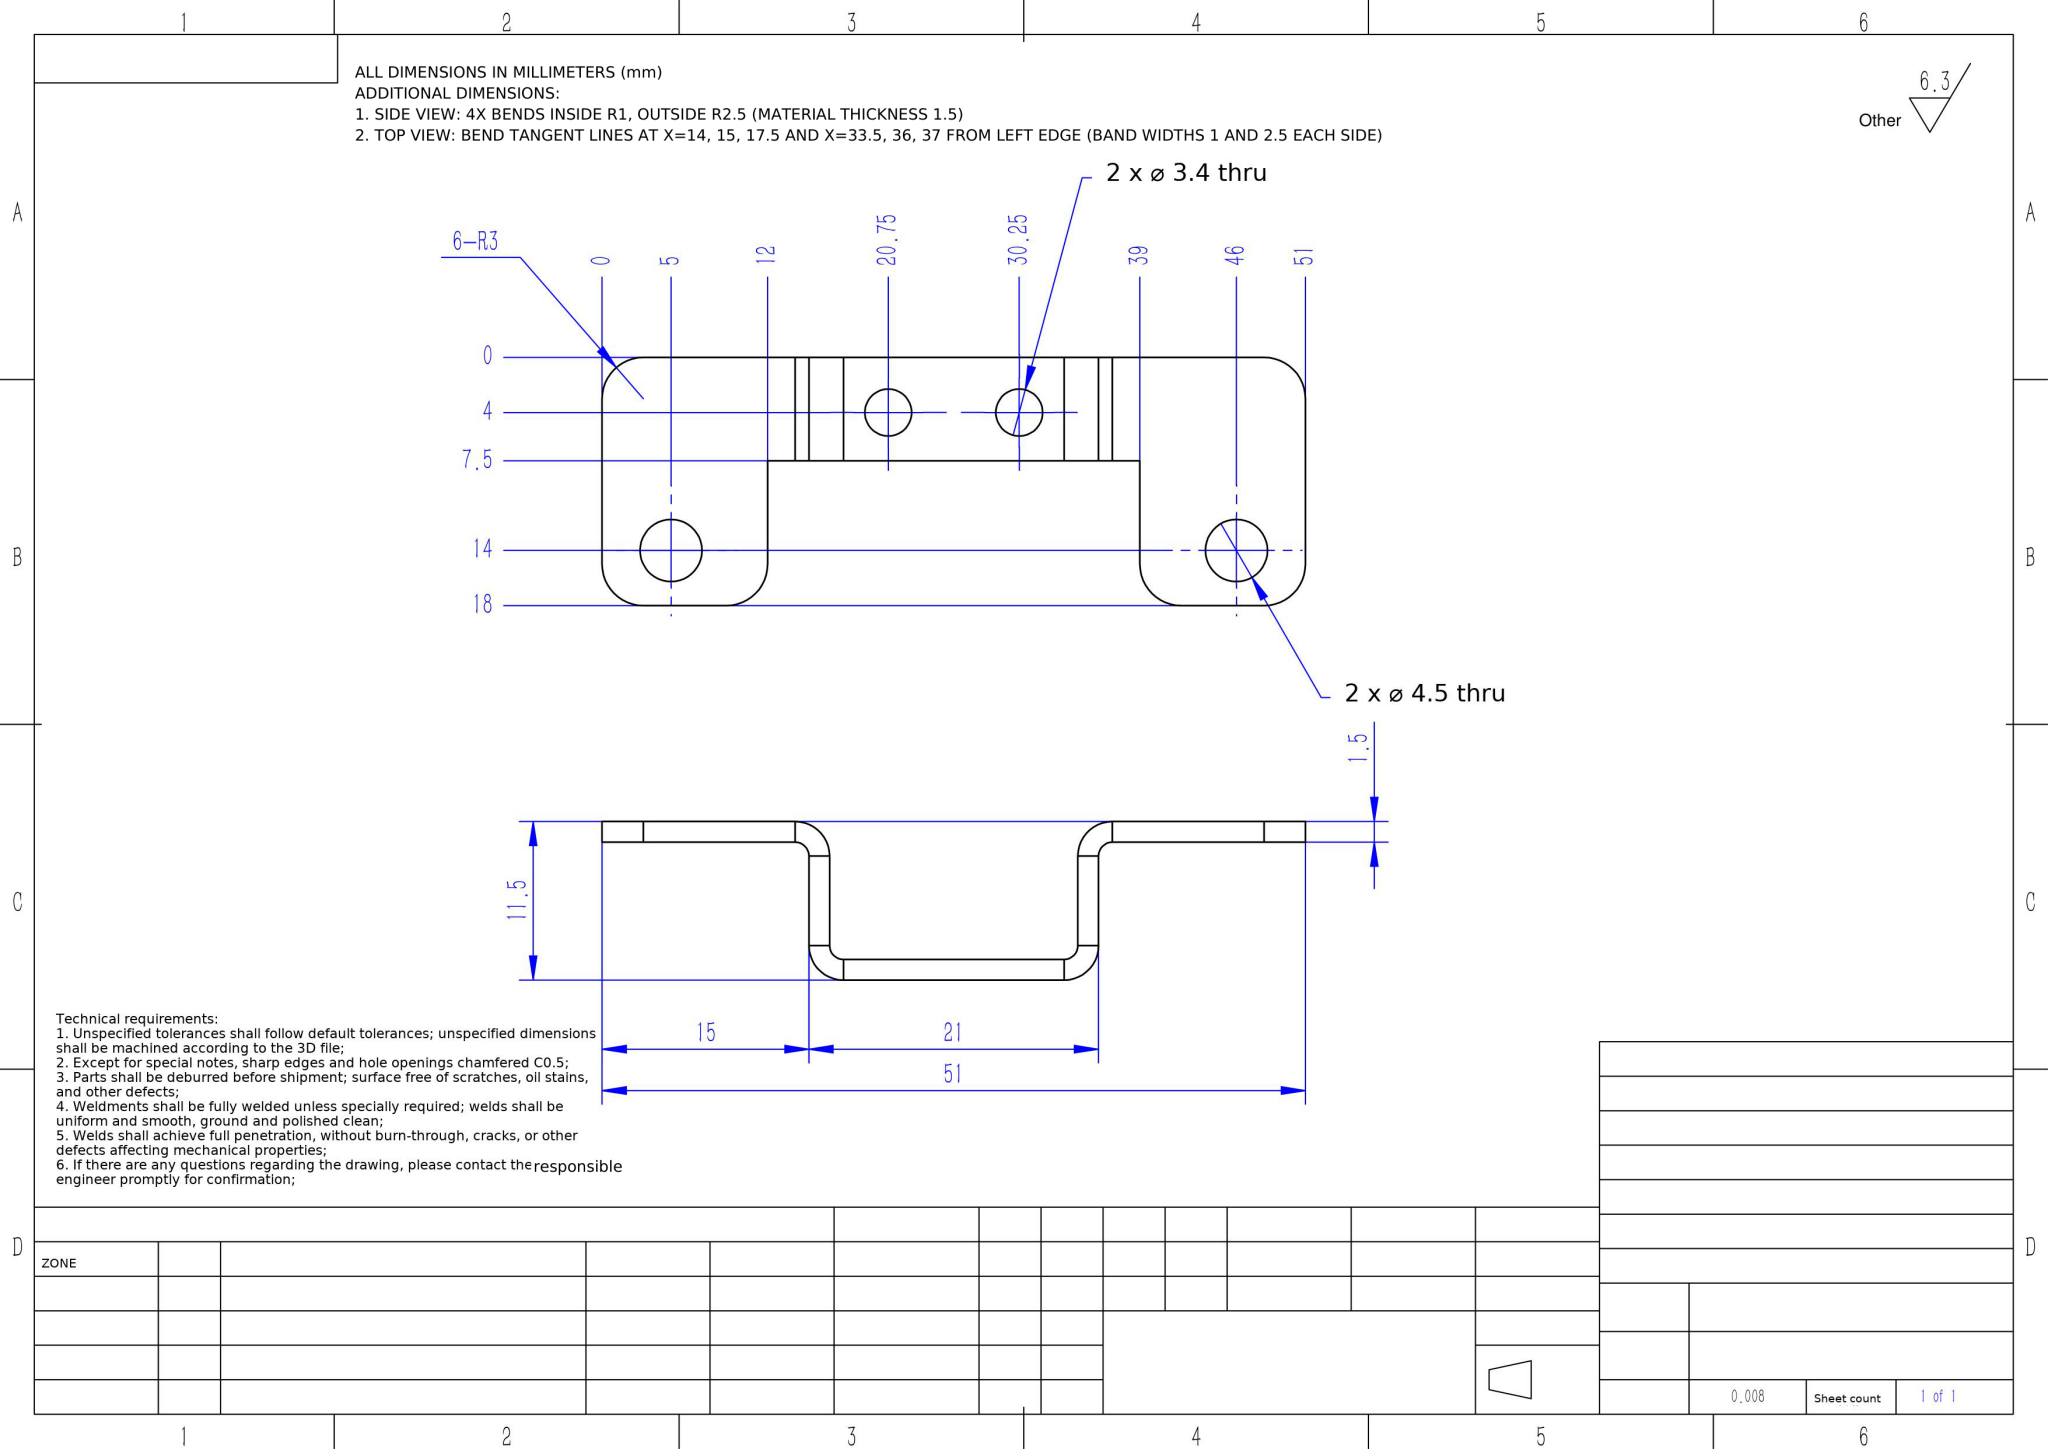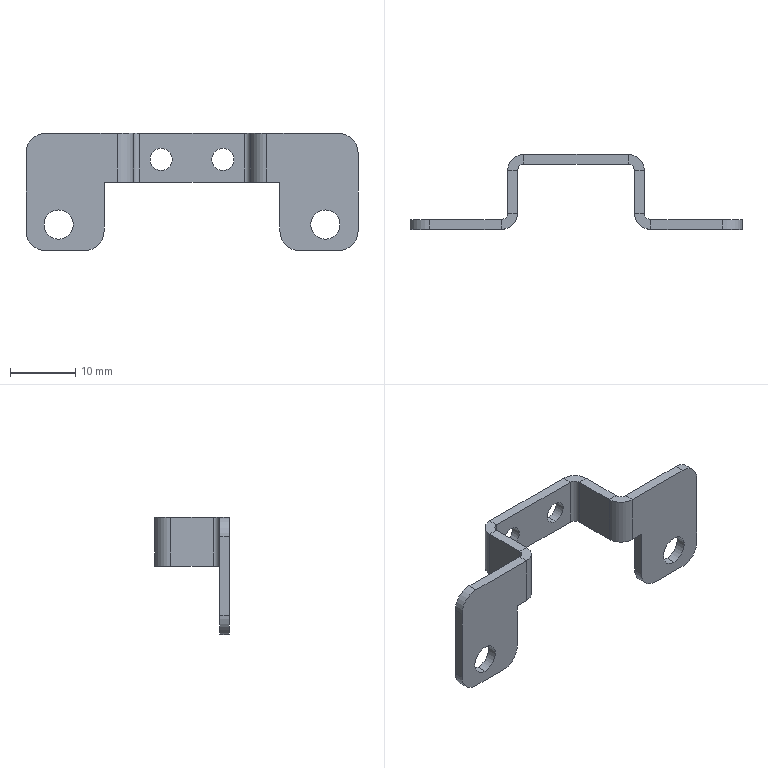Part | NX | mm | 1 solid | 56 faces | box 51 x 11.5 x 18 mm | volume 1051 mm3 | plane 34 | cylinder 22 | commonest cylinder face diameters 6 x6 4.5 x4 3.4 x4 2 x4 5 x4